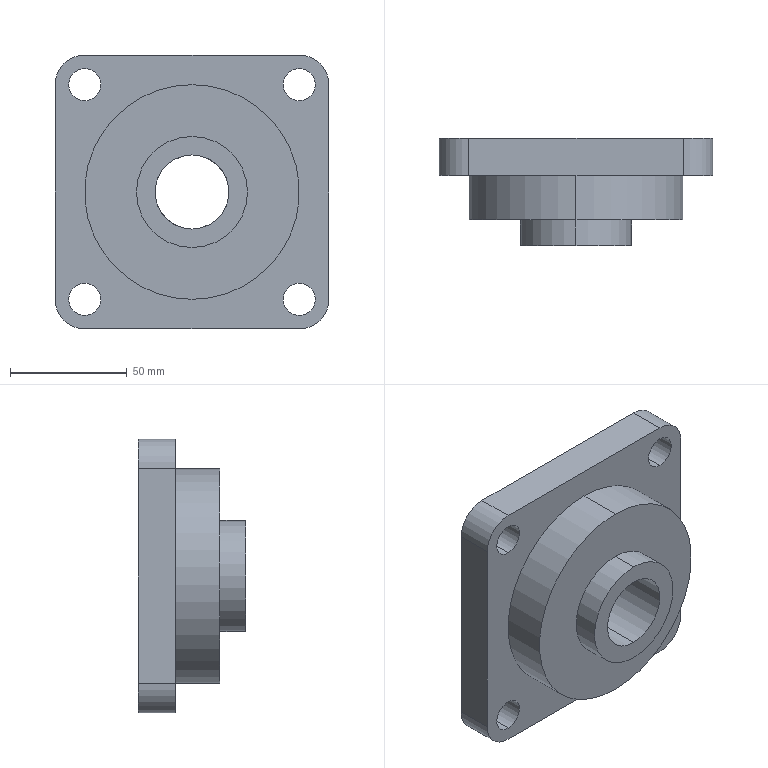Component | SolidWorks | LX-TSJ-02-1 | 1 solid | 26 faces | box 117.48 x 46.04 x 117.48 mm | volume 317559 mm3 | cylinder 18 | plane 8 | commonest cylinder face diameters 13.811 x8 25.4 x4 31.75 x2 92.075 x2 47.625 x2
STEP:
#1=COLOUR_RGB('',0.7922,0.8196,0.9333);
#2=FILL_AREA_STYLE_COLOUR('',#1);
#3=FILL_AREA_STYLE('',(#2));
#4=SURFACE_STYLE_FILL_AREA(#3);
#5=SURFACE_SIDE_STYLE('',(#4));
#6=SURFACE_STYLE_USAGE(.BOTH.,#5);
#7=PRESENTATION_STYLE_ASSIGNMENT((#6));
#8=CARTESIAN_POINT('',(-4.843,-15.157,-15.686));
#9=VERTEX_POINT('',#8);
#10=CARTESIAN_POINT('',(-4.843,-15.157,-16.936));
#11=VERTEX_POINT('',#10);
#12=CARTESIAN_POINT('',(-4.843,-15.157,-15.686));
#13=CARTESIAN_POINT('',(-4.926,-15.157,-15.686));
#14=CARTESIAN_POINT('',(-5.006,-15.157,-15.702));
#15=CARTESIAN_POINT('',(-5.159,-15.157,-15.765));
#16=CARTESIAN_POINT('',(-5.227,-15.157,-15.81));
#17=CARTESIAN_POINT('',(-5.344,-15.157,-15.928));
#18=CARTESIAN_POINT('',(-5.389,-15.157,-15.995));
#19=CARTESIAN_POINT('',(-5.453,-15.157,-16.148));
#20=CARTESIAN_POINT('',(-5.468,-15.157,-16.228));
#21=CARTESIAN_POINT('',(-5.468,-15.157,-16.394));
#22=CARTESIAN_POINT('',(-5.453,-15.157,-16.474));
#23=CARTESIAN_POINT('',(-5.389,-15.157,-16.627));
#24=CARTESIAN_POINT('',(-5.344,-15.157,-16.694));
#25=CARTESIAN_POINT('',(-5.227,-15.157,-16.811));
#26=CARTESIAN_POINT('',(-5.159,-15.157,-16.857));
#27=CARTESIAN_POINT('',(-5.006,-15.157,-16.92));
#28=CARTESIAN_POINT('',(-4.926,-15.157,-16.936));
#29=CARTESIAN_POINT('',(-4.843,-15.157,-16.936));
#30=B_SPLINE_CURVE_WITH_KNOTS('',3,(#12,#13,#14,#15,#16,#17,#18,#19,#20,#21,#22,#23,#24,#25,#26,#27,#28,#29),.UNSPECIFIED.,.F.,.F.,(4,2,2,2,2,2,2,2,4),(0.5,0.5625,0.625,0.6875,0.75,0.8125,0.875,0.9375,1.),.UNSPECIFIED.);
#31=EDGE_CURVE('',#9,#11,#30,.T.);
#32=ORIENTED_EDGE('',*,*,#31,.F.);
#33=CARTESIAN_POINT('',(-4.843,-16.969,-15.686));
#34=VERTEX_POINT('',#33);
#35=CARTESIAN_POINT('',(-4.843,-16.969,-15.686));
#36=DIRECTION('',(0.,-1.,-0.));
#37=VECTOR('',#36,39.37);
#38=LINE('',#35,#37);
#39=EDGE_CURVE('',#9,#34,#38,.T.);
#40=ORIENTED_EDGE('',*,*,#39,.T.);
#41=CARTESIAN_POINT('',(-4.843,-16.969,-16.936));
#42=VERTEX_POINT('',#41);
#43=CARTESIAN_POINT('',(-4.843,-16.969,-16.311));
#44=DIRECTION('',(0.,-1.,-0.));
#45=DIRECTION('',(0.,0.,-1.));
#46=AXIS2_PLACEMENT_3D('',#43,#44,#45);
#47=CIRCLE('',#46,0.625);
#48=EDGE_CURVE('',#34,#42,#47,.T.);
#49=ORIENTED_EDGE('',*,*,#48,.T.);
#50=CARTESIAN_POINT('',(-4.843,-16.969,-16.936));
#51=DIRECTION('',(0.,-1.,-0.));
#52=VECTOR('',#51,39.37);
#53=LINE('',#50,#52);
#54=EDGE_CURVE('',#11,#42,#53,.T.);
#55=ORIENTED_EDGE('',*,*,#54,.F.);
#56=EDGE_LOOP('',(#32,#40,#49,#55));
#57=FACE_OUTER_BOUND('',#56,.T.);
#58=CARTESIAN_POINT('',(-4.843,-16.969,-16.311));
#59=DIRECTION('',(0.,-1.,-0.));
#60=DIRECTION('',(0.,0.,-1.));
#61=AXIS2_PLACEMENT_3D('',#58,#59,#60);
#62=CYLINDRICAL_SURFACE('',#61,0.625);
#63=ADVANCED_FACE('',(#57),#62,.F.);
#64=CARTESIAN_POINT('',(-4.843,-16.532,-14.498));
#65=VERTEX_POINT('',#64);
#66=CARTESIAN_POINT('',(-4.843,-16.532,-18.123));
#67=VERTEX_POINT('',#66);
#68=CARTESIAN_POINT('',(-4.843,-16.532,-16.311));
#69=DIRECTION('',(-0.,1.,0.));
#70=DIRECTION('',(-0.,-0.,1.));
#71=AXIS2_PLACEMENT_3D('',#68,#69,#70);
#72=CIRCLE('',#71,1.813);
#73=EDGE_CURVE('',#65,#67,#72,.T.);
#74=ORIENTED_EDGE('',*,*,#73,.T.);
#75=CARTESIAN_POINT('',(-4.843,-15.782,-18.123));
#76=VERTEX_POINT('',#75);
#77=CARTESIAN_POINT('',(-4.843,-16.532,-18.123));
#78=DIRECTION('',(-0.,1.,0.));
#79=VECTOR('',#78,39.37);
#80=LINE('',#77,#79);
#81=EDGE_CURVE('',#67,#76,#80,.T.);
#82=ORIENTED_EDGE('',*,*,#81,.T.);
#83=CARTESIAN_POINT('',(-4.843,-15.782,-14.498));
#84=VERTEX_POINT('',#83);
#85=CARTESIAN_POINT('',(-4.843,-15.782,-16.311));
#86=DIRECTION('',(-0.,1.,0.));
#87=DIRECTION('',(-0.,-0.,1.));
#88=AXIS2_PLACEMENT_3D('',#85,#86,#87);
#89=CIRCLE('',#88,1.813);
#90=EDGE_CURVE('',#84,#76,#89,.T.);
#91=ORIENTED_EDGE('',*,*,#90,.F.);
#92=CARTESIAN_POINT('',(-4.843,-16.532,-14.498));
#93=DIRECTION('',(-0.,1.,0.));
#94=VECTOR('',#93,39.37);
#95=LINE('',#92,#94);
#96=EDGE_CURVE('',#65,#84,#95,.T.);
#97=ORIENTED_EDGE('',*,*,#96,.F.);
#98=EDGE_LOOP('',(#74,#82,#91,#97));
#99=FACE_OUTER_BOUND('',#98,.T.);
#100=CARTESIAN_POINT('',(-4.843,-16.532,-16.311));
#101=DIRECTION('',(-0.,1.,0.));
#102=DIRECTION('',(-0.,-0.,1.));
#103=AXIS2_PLACEMENT_3D('',#100,#101,#102);
#104=CYLINDRICAL_SURFACE('',#103,1.813);
#105=ADVANCED_FACE('',(#99),#104,.T.);
#106=CARTESIAN_POINT('',(-6.656,-15.157,-14.77));
#107=VERTEX_POINT('',#106);
#108=CARTESIAN_POINT('',(-6.656,-15.157,-14.227));
#109=VERTEX_POINT('',#108);
#110=CARTESIAN_POINT('',(-6.656,-15.157,-14.498));
#111=DIRECTION('',(-0.,1.,0.));
#112=DIRECTION('',(0.,0.,-1.));
#113=AXIS2_PLACEMENT_3D('',#110,#111,#112);
#114=CIRCLE('',#113,0.2719);
#115=EDGE_CURVE('',#107,#109,#114,.T.);
#116=ORIENTED_EDGE('',*,*,#115,.T.);
#117=CARTESIAN_POINT('',(-6.656,-15.782,-14.227));
#118=VERTEX_POINT('',#117);
#119=CARTESIAN_POINT('',(-6.656,-15.782,-14.227));
#120=DIRECTION('',(0.,-1.,-0.));
#121=VECTOR('',#120,39.37);
#122=LINE('',#119,#121);
#123=EDGE_CURVE('',#109,#118,#122,.T.);
#124=ORIENTED_EDGE('',*,*,#123,.T.);
#125=CARTESIAN_POINT('',(-6.656,-15.782,-14.77));
#126=VERTEX_POINT('',#125);
#127=CARTESIAN_POINT('',(-6.656,-15.782,-14.498));
#128=DIRECTION('',(-0.,1.,0.));
#129=DIRECTION('',(0.,0.,-1.));
#130=AXIS2_PLACEMENT_3D('',#127,#128,#129);
#131=CIRCLE('',#130,0.2719);
#132=EDGE_CURVE('',#126,#118,#131,.T.);
#133=ORIENTED_EDGE('',*,*,#132,.F.);
#134=CARTESIAN_POINT('',(-6.656,-15.782,-14.77));
#135=DIRECTION('',(0.,-1.,-0.));
#136=VECTOR('',#135,39.37);
#137=LINE('',#134,#136);
#138=EDGE_CURVE('',#107,#126,#137,.T.);
#139=ORIENTED_EDGE('',*,*,#138,.F.);
#140=EDGE_LOOP('',(#116,#124,#133,#139));
#141=FACE_OUTER_BOUND('',#140,.T.);
#142=CARTESIAN_POINT('',(-6.656,-15.782,-14.498));
#143=DIRECTION('',(0.,-1.,-0.));
#144=DIRECTION('',(0.,0.,-1.));
#145=AXIS2_PLACEMENT_3D('',#142,#143,#144);
#146=CYLINDRICAL_SURFACE('',#145,0.2719);
#147=ADVANCED_FACE('',(#141),#146,.F.);
#148=CARTESIAN_POINT('',(-6.656,-15.157,-18.395));
#149=VERTEX_POINT('',#148);
#150=CARTESIAN_POINT('',(-6.656,-15.157,-17.852));
#151=VERTEX_POINT('',#150);
#152=CARTESIAN_POINT('',(-6.656,-15.157,-18.123));
#153=DIRECTION('',(-0.,1.,0.));
#154=DIRECTION('',(0.,0.,-1.));
#155=AXIS2_PLACEMENT_3D('',#152,#153,#154);
#156=CIRCLE('',#155,0.2719);
#157=EDGE_CURVE('',#149,#151,#156,.T.);
#158=ORIENTED_EDGE('',*,*,#157,.T.);
#159=CARTESIAN_POINT('',(-6.656,-15.782,-17.852));
#160=VERTEX_POINT('',#159);
#161=CARTESIAN_POINT('',(-6.656,-15.782,-17.852));
#162=DIRECTION('',(0.,-1.,-0.));
#163=VECTOR('',#162,39.37);
#164=LINE('',#161,#163);
#165=EDGE_CURVE('',#151,#160,#164,.T.);
#166=ORIENTED_EDGE('',*,*,#165,.T.);
#167=CARTESIAN_POINT('',(-6.656,-15.782,-18.395));
#168=VERTEX_POINT('',#167);
#169=CARTESIAN_POINT('',(-6.656,-15.782,-18.123));
#170=DIRECTION('',(-0.,1.,0.));
#171=DIRECTION('',(0.,0.,-1.));
#172=AXIS2_PLACEMENT_3D('',#169,#170,#171);
#173=CIRCLE('',#172,0.2719);
#174=EDGE_CURVE('',#168,#160,#173,.T.);
#175=ORIENTED_EDGE('',*,*,#174,.F.);
#176=CARTESIAN_POINT('',(-6.656,-15.782,-18.395));
#177=DIRECTION('',(0.,-1.,-0.));
#178=VECTOR('',#177,39.37);
#179=LINE('',#176,#178);
#180=EDGE_CURVE('',#149,#168,#179,.T.);
#181=ORIENTED_EDGE('',*,*,#180,.F.);
#182=EDGE_LOOP('',(#158,#166,#175,#181));
#183=FACE_OUTER_BOUND('',#182,.T.);
#184=CARTESIAN_POINT('',(-6.656,-15.782,-18.123));
#185=DIRECTION('',(0.,-1.,-0.));
#186=DIRECTION('',(0.,0.,-1.));
#187=AXIS2_PLACEMENT_3D('',#184,#185,#186);
#188=CYLINDRICAL_SURFACE('',#187,0.2719);
#189=ADVANCED_FACE('',(#183),#188,.F.);
#190=CARTESIAN_POINT('',(-3.031,-15.157,-14.77));
#191=VERTEX_POINT('',#190);
#192=CARTESIAN_POINT('',(-3.031,-15.157,-14.227));
#193=VERTEX_POINT('',#192);
#194=CARTESIAN_POINT('',(-3.031,-15.157,-14.498));
#195=DIRECTION('',(-0.,1.,0.));
#196=DIRECTION('',(0.,0.,-1.));
#197=AXIS2_PLACEMENT_3D('',#194,#195,#196);
#198=CIRCLE('',#197,0.2719);
#199=EDGE_CURVE('',#191,#193,#198,.T.);
#200=ORIENTED_EDGE('',*,*,#199,.T.);
#201=CARTESIAN_POINT('',(-3.031,-15.782,-14.227));
#202=VERTEX_POINT('',#201);
#203=CARTESIAN_POINT('',(-3.031,-15.782,-14.227));
#204=DIRECTION('',(0.,-1.,-0.));
#205=VECTOR('',#204,39.37);
#206=LINE('',#203,#205);
#207=EDGE_CURVE('',#193,#202,#206,.T.);
#208=ORIENTED_EDGE('',*,*,#207,.T.);
#209=CARTESIAN_POINT('',(-3.031,-15.782,-14.77));
#210=VERTEX_POINT('',#209);
#211=CARTESIAN_POINT('',(-3.031,-15.782,-14.498));
#212=DIRECTION('',(-0.,1.,0.));
#213=DIRECTION('',(0.,0.,-1.));
#214=AXIS2_PLACEMENT_3D('',#211,#212,#213);
#215=CIRCLE('',#214,0.2719);
#216=EDGE_CURVE('',#210,#202,#215,.T.);
#217=ORIENTED_EDGE('',*,*,#216,.F.);
#218=CARTESIAN_POINT('',(-3.031,-15.782,-14.77));
#219=DIRECTION('',(0.,-1.,-0.));
#220=VECTOR('',#219,39.37);
#221=LINE('',#218,#220);
#222=EDGE_CURVE('',#191,#210,#221,.T.);
#223=ORIENTED_EDGE('',*,*,#222,.F.);
#224=EDGE_LOOP('',(#200,#208,#217,#223));
#225=FACE_OUTER_BOUND('',#224,.T.);
#226=CARTESIAN_POINT('',(-3.031,-15.782,-14.498));
#227=DIRECTION('',(0.,-1.,-0.));
#228=DIRECTION('',(0.,0.,-1.));
#229=AXIS2_PLACEMENT_3D('',#226,#227,#228);
#230=CYLINDRICAL_SURFACE('',#229,0.2719);
#231=ADVANCED_FACE('',(#225),#230,.F.);
#232=CARTESIAN_POINT('',(-3.031,-15.157,-18.395));
#233=VERTEX_POINT('',#232);
#234=CARTESIAN_POINT('',(-3.031,-15.157,-17.852));
#235=VERTEX_POINT('',#234);
#236=CARTESIAN_POINT('',(-3.031,-15.157,-18.123));
#237=DIRECTION('',(-0.,1.,0.));
#238=DIRECTION('',(0.,0.,-1.));
#239=AXIS2_PLACEMENT_3D('',#236,#237,#238);
#240=CIRCLE('',#239,0.2719);
#241=EDGE_CURVE('',#233,#235,#240,.T.);
#242=ORIENTED_EDGE('',*,*,#241,.T.);
#243=CARTESIAN_POINT('',(-3.031,-15.782,-17.852));
#244=VERTEX_POINT('',#243);
#245=CARTESIAN_POINT('',(-3.031,-15.782,-17.852));
#246=DIRECTION('',(0.,-1.,-0.));
#247=VECTOR('',#246,39.37);
#248=LINE('',#245,#247);
#249=EDGE_CURVE('',#235,#244,#248,.T.);
#250=ORIENTED_EDGE('',*,*,#249,.T.);
#251=CARTESIAN_POINT('',(-3.031,-15.782,-18.395));
#252=VERTEX_POINT('',#251);
#253=CARTESIAN_POINT('',(-3.031,-15.782,-18.123));
#254=DIRECTION('',(-0.,1.,0.));
#255=DIRECTION('',(0.,0.,-1.));
#256=AXIS2_PLACEMENT_3D('',#253,#254,#255);
#257=CIRCLE('',#256,0.2719);
#258=EDGE_CURVE('',#252,#244,#257,.T.);
#259=ORIENTED_EDGE('',*,*,#258,.F.);
#260=CARTESIAN_POINT('',(-3.031,-15.782,-18.395));
#261=DIRECTION('',(0.,-1.,-0.));
#262=VECTOR('',#261,39.37);
#263=LINE('',#260,#262);
#264=EDGE_CURVE('',#233,#252,#263,.T.);
#265=ORIENTED_EDGE('',*,*,#264,.F.);
#266=EDGE_LOOP('',(#242,#250,#259,#265));
#267=FACE_OUTER_BOUND('',#266,.T.);
#268=CARTESIAN_POINT('',(-3.031,-15.782,-18.123));
#269=DIRECTION('',(0.,-1.,-0.));
#270=DIRECTION('',(0.,0.,-1.));
#271=AXIS2_PLACEMENT_3D('',#268,#269,#270);
#272=CYLINDRICAL_SURFACE('',#271,0.2719);
#273=ADVANCED_FACE('',(#267),#272,.F.);
#274=CARTESIAN_POINT('',(-4.843,-16.969,-17.248));
#275=VERTEX_POINT('',#274);
#276=CARTESIAN_POINT('',(-4.843,-16.969,-15.373));
#277=VERTEX_POINT('',#276);
#278=CARTESIAN_POINT('',(-4.843,-16.969,-16.311));
#279=DIRECTION('',(0.,-1.,-0.));
#280=DIRECTION('',(0.,0.,-1.));
#281=AXIS2_PLACEMENT_3D('',#278,#279,#280);
#282=CIRCLE('',#281,0.9375);
#283=EDGE_CURVE('',#275,#277,#282,.T.);
#284=ORIENTED_EDGE('',*,*,#283,.F.);
#285=CARTESIAN_POINT('',(-4.843,-16.532,-17.248));
#286=VERTEX_POINT('',#285);
#287=CARTESIAN_POINT('',(-4.843,-16.969,-17.248));
#288=DIRECTION('',(-0.,1.,0.));
#289=VECTOR('',#288,39.37);
#290=LINE('',#287,#289);
#291=EDGE_CURVE('',#275,#286,#290,.T.);
#292=ORIENTED_EDGE('',*,*,#291,.T.);
#293=CARTESIAN_POINT('',(-4.843,-16.532,-15.373));
#294=VERTEX_POINT('',#293);
#295=CARTESIAN_POINT('',(-4.843,-16.532,-16.311));
#296=DIRECTION('',(-0.,1.,0.));
#297=DIRECTION('',(0.,0.,-1.));
#298=AXIS2_PLACEMENT_3D('',#295,#296,#297);
#299=CIRCLE('',#298,0.9375);
#300=EDGE_CURVE('',#294,#286,#299,.T.);
#301=ORIENTED_EDGE('',*,*,#300,.F.);
#302=CARTESIAN_POINT('',(-4.843,-16.969,-15.373));
#303=DIRECTION('',(-0.,1.,0.));
#304=VECTOR('',#303,39.37);
#305=LINE('',#302,#304);
#306=EDGE_CURVE('',#277,#294,#305,.T.);
#307=ORIENTED_EDGE('',*,*,#306,.F.);
#308=EDGE_LOOP('',(#284,#292,#301,#307));
#309=FACE_OUTER_BOUND('',#308,.T.);
#310=CARTESIAN_POINT('',(-4.843,-16.969,-16.311));
#311=DIRECTION('',(-0.,1.,0.));
#312=DIRECTION('',(0.,-0.,1.));
#313=AXIS2_PLACEMENT_3D('',#310,#311,#312);
#314=CYLINDRICAL_SURFACE('',#313,0.9375);
#315=ADVANCED_FACE('',(#309),#314,.T.);
#316=ORIENTED_EDGE('',*,*,#291,.F.);
#317=CARTESIAN_POINT('',(-4.843,-16.969,-16.311));
#318=DIRECTION('',(0.,-1.,-0.));
#319=DIRECTION('',(0.,0.,-1.));
#320=AXIS2_PLACEMENT_3D('',#317,#318,#319);
#321=CIRCLE('',#320,0.9375);
#322=EDGE_CURVE('',#277,#275,#321,.T.);
#323=ORIENTED_EDGE('',*,*,#322,.F.);
#324=ORIENTED_EDGE('',*,*,#306,.T.);
#325=CARTESIAN_POINT('',(-4.843,-16.532,-16.311));
#326=DIRECTION('',(-0.,1.,0.));
#327=DIRECTION('',(0.,0.,-1.));
#328=AXIS2_PLACEMENT_3D('',#325,#326,#327);
#329=CIRCLE('',#328,0.9375);
#330=EDGE_CURVE('',#286,#294,#329,.T.);
#331=ORIENTED_EDGE('',*,*,#330,.F.);
#332=EDGE_LOOP('',(#316,#323,#324,#331));
#333=FACE_OUTER_BOUND('',#332,.T.);
#334=CARTESIAN_POINT('',(-4.843,-16.969,-16.311));
#335=DIRECTION('',(-0.,1.,0.));
#336=DIRECTION('',(0.,-0.,1.));
#337=AXIS2_PLACEMENT_3D('',#334,#335,#336);
#338=CYLINDRICAL_SURFACE('',#337,0.9375);
#339=ADVANCED_FACE('',(#333),#338,.T.);
#340=CARTESIAN_POINT('',(-4.843,-15.157,-16.936));
#341=CARTESIAN_POINT('',(-4.761,-15.157,-16.936));
#342=CARTESIAN_POINT('',(-4.681,-15.157,-16.92));
#343=CARTESIAN_POINT('',(-4.528,-15.157,-16.857));
#344=CARTESIAN_POINT('',(-4.46,-15.157,-16.811));
#345=CARTESIAN_POINT('',(-4.343,-15.157,-16.694));
#346=CARTESIAN_POINT('',(-4.298,-15.157,-16.627));
#347=CARTESIAN_POINT('',(-4.234,-15.157,-16.474));
#348=CARTESIAN_POINT('',(-4.218,-15.157,-16.394));
#349=CARTESIAN_POINT('',(-4.218,-15.157,-16.228));
#350=CARTESIAN_POINT('',(-4.234,-15.157,-16.148));
#351=CARTESIAN_POINT('',(-4.298,-15.157,-15.995));
#352=CARTESIAN_POINT('',(-4.343,-15.157,-15.928));
#353=CARTESIAN_POINT('',(-4.46,-15.157,-15.81));
#354=CARTESIAN_POINT('',(-4.528,-15.157,-15.765));
#355=CARTESIAN_POINT('',(-4.681,-15.157,-15.702));
#356=CARTESIAN_POINT('',(-4.761,-15.157,-15.686));
#357=CARTESIAN_POINT('',(-4.843,-15.157,-15.686));
#358=B_SPLINE_CURVE_WITH_KNOTS('',3,(#340,#341,#342,#343,#344,#345,#346,#347,#348,#349,#350,#351,#352,#353,#354,#355,#356,#357),.UNSPECIFIED.,.F.,.F.,(4,2,2,2,2,2,2,2,4),(0.,0.0625,0.125,0.1875,0.25,0.3125,0.375,0.4375,0.5),.UNSPECIFIED.);
#359=EDGE_CURVE('',#11,#9,#358,.T.);
#360=ORIENTED_EDGE('',*,*,#359,.T.);
#361=ORIENTED_EDGE('',*,*,#31,.T.);
#362=EDGE_LOOP('',(#360,#361));
#363=FACE_BOUND('',#362,.T.);
#364=CARTESIAN_POINT('',(-3.031,-15.157,-18.623));
#365=VERTEX_POINT('',#364);
#366=CARTESIAN_POINT('',(-2.531,-15.157,-18.123));
#367=VERTEX_POINT('',#366);
#368=CARTESIAN_POINT('',(-3.031,-15.157,-18.123));
#369=DIRECTION('',(0.,-1.,-0.));
#370=DIRECTION('',(0.,0.,-1.));
#371=AXIS2_PLACEMENT_3D('',#368,#369,#370);
#372=CIRCLE('',#371,0.5);
#373=EDGE_CURVE('',#365,#367,#372,.T.);
#374=ORIENTED_EDGE('',*,*,#373,.F.);
#375=CARTESIAN_POINT('',(-6.656,-15.157,-18.623));
#376=VERTEX_POINT('',#375);
#377=CARTESIAN_POINT('',(-7.156,-15.157,-18.623));
#378=DIRECTION('',(1.,0.,0.));
#379=VECTOR('',#378,39.37);
#380=LINE('',#377,#379);
#381=EDGE_CURVE('',#376,#365,#380,.T.);
#382=ORIENTED_EDGE('',*,*,#381,.F.);
#383=CARTESIAN_POINT('',(-7.156,-15.157,-18.123));
#384=VERTEX_POINT('',#383);
#385=CARTESIAN_POINT('',(-6.656,-15.157,-18.123));
#386=DIRECTION('',(0.,-1.,-0.));
#387=DIRECTION('',(0.,-0.,1.));
#388=AXIS2_PLACEMENT_3D('',#385,#386,#387);
#389=CIRCLE('',#388,0.5);
#390=EDGE_CURVE('',#384,#376,#389,.T.);
#391=ORIENTED_EDGE('',*,*,#390,.F.);
#392=CARTESIAN_POINT('',(-7.156,-15.157,-14.498));
#393=VERTEX_POINT('',#392);
#394=CARTESIAN_POINT('',(-7.156,-15.157,-18.623));
#395=DIRECTION('',(0.,0.,-1.));
#396=VECTOR('',#395,39.37);
#397=LINE('',#394,#396);
#398=EDGE_CURVE('',#393,#384,#397,.T.);
#399=ORIENTED_EDGE('',*,*,#398,.F.);
#400=CARTESIAN_POINT('',(-6.656,-15.157,-13.998));
#401=VERTEX_POINT('',#400);
#402=CARTESIAN_POINT('',(-6.656,-15.157,-14.498));
#403=DIRECTION('',(0.,-1.,-0.));
#404=DIRECTION('',(0.,0.,-1.));
#405=AXIS2_PLACEMENT_3D('',#402,#403,#404);
#406=CIRCLE('',#405,0.5);
#407=EDGE_CURVE('',#401,#393,#406,.T.);
#408=ORIENTED_EDGE('',*,*,#407,.F.);
#409=CARTESIAN_POINT('',(-3.031,-15.157,-13.998));
#410=VERTEX_POINT('',#409);
#411=CARTESIAN_POINT('',(-7.156,-15.157,-13.998));
#412=DIRECTION('',(-1.,-0.,-0.));
#413=VECTOR('',#412,39.37);
#414=LINE('',#411,#413);
#415=EDGE_CURVE('',#410,#401,#414,.T.);
#416=ORIENTED_EDGE('',*,*,#415,.F.);
#417=CARTESIAN_POINT('',(-2.531,-15.157,-14.498));
#418=VERTEX_POINT('',#417);
#419=CARTESIAN_POINT('',(-3.031,-15.157,-14.498));
#420=DIRECTION('',(0.,-1.,-0.));
#421=DIRECTION('',(0.,0.,-1.));
#422=AXIS2_PLACEMENT_3D('',#419,#420,#421);
#423=CIRCLE('',#422,0.5);
#424=EDGE_CURVE('',#418,#410,#423,.T.);
#425=ORIENTED_EDGE('',*,*,#424,.F.);
#426=CARTESIAN_POINT('',(-2.531,-15.157,-18.623));
#427=DIRECTION('',(-0.,-0.,1.));
#428=VECTOR('',#427,39.37);
#429=LINE('',#426,#428);
#430=EDGE_CURVE('',#367,#418,#429,.T.);
#431=ORIENTED_EDGE('',*,*,#430,.F.);
#432=EDGE_LOOP('',(#374,#382,#391,#399,#408,#416,#425,#431));
#433=FACE_OUTER_BOUND('',#432,.T.);
#434=ORIENTED_EDGE('',*,*,#115,.F.);
#435=CARTESIAN_POINT('',(-6.656,-15.157,-14.498));
#436=DIRECTION('',(-0.,1.,0.));
#437=DIRECTION('',(0.,0.,-1.));
#438=AXIS2_PLACEMENT_3D('',#435,#436,#437);
#439=CIRCLE('',#438,0.2719);
#440=EDGE_CURVE('',#109,#107,#439,.T.);
#441=ORIENTED_EDGE('',*,*,#440,.F.);
#442=EDGE_LOOP('',(#434,#441));
#443=FACE_BOUND('',#442,.T.);
#444=ORIENTED_EDGE('',*,*,#157,.F.);
#445=CARTESIAN_POINT('',(-6.656,-15.157,-18.123));
#446=DIRECTION('',(-0.,1.,0.));
#447=DIRECTION('',(0.,0.,-1.));
#448=AXIS2_PLACEMENT_3D('',#445,#446,#447);
#449=CIRCLE('',#448,0.2719);
#450=EDGE_CURVE('',#151,#149,#449,.T.);
#451=ORIENTED_EDGE('',*,*,#450,.F.);
#452=EDGE_LOOP('',(#444,#451));
#453=FACE_BOUND('',#452,.T.);
#454=ORIENTED_EDGE('',*,*,#199,.F.);
#455=CARTESIAN_POINT('',(-3.031,-15.157,-14.498));
#456=DIRECTION('',(-0.,1.,0.));
#457=DIRECTION('',(0.,0.,-1.));
#458=AXIS2_PLACEMENT_3D('',#455,#456,#457);
#459=CIRCLE('',#458,0.2719);
#460=EDGE_CURVE('',#193,#191,#459,.T.);
#461=ORIENTED_EDGE('',*,*,#460,.F.);
#462=EDGE_LOOP('',(#454,#461));
#463=FACE_BOUND('',#462,.T.);
#464=ORIENTED_EDGE('',*,*,#241,.F.);
#465=CARTESIAN_POINT('',(-3.031,-15.157,-18.123));
#466=DIRECTION('',(-0.,1.,0.));
#467=DIRECTION('',(0.,0.,-1.));
#468=AXIS2_PLACEMENT_3D('',#465,#466,#467);
#469=CIRCLE('',#468,0.2719);
#470=EDGE_CURVE('',#235,#233,#469,.T.);
#471=ORIENTED_EDGE('',*,*,#470,.F.);
#472=EDGE_LOOP('',(#464,#471));
#473=FACE_BOUND('',#472,.T.);
#474=CARTESIAN_POINT('',(-7.156,-15.157,-18.623));
#475=DIRECTION('',(0.,-1.,-0.));
#476=DIRECTION('',(0.,0.,-1.));
#477=AXIS2_PLACEMENT_3D('',#474,#475,#476);
#478=PLANE('',#477);
#479=ADVANCED_FACE('',(#363,#433,#443,#453,#463,#473),#478,.F.);
#480=ORIENTED_EDGE('',*,*,#249,.F.);
#481=ORIENTED_EDGE('',*,*,#470,.T.);
#482=ORIENTED_EDGE('',*,*,#264,.T.);
#483=CARTESIAN_POINT('',(-3.031,-15.782,-18.123));
#484=DIRECTION('',(-0.,1.,0.));
#485=DIRECTION('',(0.,0.,-1.));
#486=AXIS2_PLACEMENT_3D('',#483,#484,#485);
#487=CIRCLE('',#486,0.2719);
#488=EDGE_CURVE('',#244,#252,#487,.T.);
#489=ORIENTED_EDGE('',*,*,#488,.F.);
#490=EDGE_LOOP('',(#480,#481,#482,#489));
#491=FACE_OUTER_BOUND('',#490,.T.);
#492=CARTESIAN_POINT('',(-3.031,-15.782,-18.123));
#493=DIRECTION('',(0.,-1.,-0.));
#494=DIRECTION('',(0.,0.,-1.));
#495=AXIS2_PLACEMENT_3D('',#492,#493,#494);
#496=CYLINDRICAL_SURFACE('',#495,0.2719);
#497=ADVANCED_FACE('',(#491),#496,.F.);
#498=ORIENTED_EDGE('',*,*,#207,.F.);
#499=ORIENTED_EDGE('',*,*,#460,.T.);
#500=ORIENTED_EDGE('',*,*,#222,.T.);
#501=CARTESIAN_POINT('',(-3.031,-15.782,-14.498));
#502=DIRECTION('',(-0.,1.,0.));
#503=DIRECTION('',(0.,0.,-1.));
#504=AXIS2_PLACEMENT_3D('',#501,#502,#503);
#505=CIRCLE('',#504,0.2719);
#506=EDGE_CURVE('',#202,#210,#505,.T.);
#507=ORIENTED_EDGE('',*,*,#506,.F.);
#508=EDGE_LOOP('',(#498,#499,#500,#507));
#509=FACE_OUTER_BOUND('',#508,.T.);
#510=CARTESIAN_POINT('',(-3.031,-15.782,-14.498));
#511=DIRECTION('',(0.,-1.,-0.));
#512=DIRECTION('',(0.,0.,-1.));
#513=AXIS2_PLACEMENT_3D('',#510,#511,#512);
#514=CYLINDRICAL_SURFACE('',#513,0.2719);
#515=ADVANCED_FACE('',(#509),#514,.F.);
#516=ORIENTED_EDGE('',*,*,#165,.F.);
#517=ORIENTED_EDGE('',*,*,#450,.T.);
#518=ORIENTED_EDGE('',*,*,#180,.T.);
#519=CARTESIAN_POINT('',(-6.656,-15.782,-18.123));
#520=DIRECTION('',(-0.,1.,0.));
#521=DIRECTION('',(0.,0.,-1.));
#522=AXIS2_PLACEMENT_3D('',#519,#520,#521);
#523=CIRCLE('',#522,0.2719);
#524=EDGE_CURVE('',#160,#168,#523,.T.);
#525=ORIENTED_EDGE('',*,*,#524,.F.);
#526=EDGE_LOOP('',(#516,#517,#518,#525));
#527=FACE_OUTER_BOUND('',#526,.T.);
#528=CARTESIAN_POINT('',(-6.656,-15.782,-18.123));
#529=DIRECTION('',(0.,-1.,-0.));
#530=DIRECTION('',(0.,0.,-1.));
#531=AXIS2_PLACEMENT_3D('',#528,#529,#530);
#532=CYLINDRICAL_SURFACE('',#531,0.2719);
#533=ADVANCED_FACE('',(#527),#532,.F.);
#534=ORIENTED_EDGE('',*,*,#123,.F.);
#535=ORIENTED_EDGE('',*,*,#440,.T.);
#536=ORIENTED_EDGE('',*,*,#138,.T.);
#537=CARTESIAN_POINT('',(-6.656,-15.782,-14.498));
#538=DIRECTION('',(-0.,1.,0.));
#539=DIRECTION('',(0.,0.,-1.));
#540=AXIS2_PLACEMENT_3D('',#537,#538,#539);
#541=CIRCLE('',#540,0.2719);
#542=EDGE_CURVE('',#118,#126,#541,.T.);
#543=ORIENTED_EDGE('',*,*,#542,.F.);
#544=EDGE_LOOP('',(#534,#535,#536,#543));
#545=FACE_OUTER_BOUND('',#544,.T.);
#546=CARTESIAN_POINT('',(-6.656,-15.782,-14.498));
#547=DIRECTION('',(0.,-1.,-0.));
#548=DIRECTION('',(0.,0.,-1.));
#549=AXIS2_PLACEMENT_3D('',#546,#547,#548);
#550=CYLINDRICAL_SURFACE('',#549,0.2719);
#551=ADVANCED_FACE('',(#545),#550,.F.);
#552=CARTESIAN_POINT('',(-7.156,-15.782,-14.498));
#553=VERTEX_POINT('',#552);
#554=CARTESIAN_POINT('',(-6.656,-15.782,-13.998));
#555=VERTEX_POINT('',#554);
#556=CARTESIAN_POINT('',(-6.656,-15.782,-14.498));
#557=DIRECTION('',(-0.,1.,0.));
#558=DIRECTION('',(0.,0.,-1.));
#559=AXIS2_PLACEMENT_3D('',#556,#557,#558);
#560=CIRCLE('',#559,0.5);
#561=EDGE_CURVE('',#553,#555,#560,.T.);
#562=ORIENTED_EDGE('',*,*,#561,.T.);
#563=CARTESIAN_POINT('',(-6.656,-15.157,-13.998));
#564=DIRECTION('',(-0.,1.,0.));
#565=VECTOR('',#564,39.37);
#566=LINE('',#563,#565);
#567=EDGE_CURVE('',#555,#401,#566,.T.);
#568=ORIENTED_EDGE('',*,*,#567,.T.);
#569=ORIENTED_EDGE('',*,*,#407,.T.);
#570=CARTESIAN_POINT('',(-7.156,-15.157,-14.498));
#571=DIRECTION('',(0.,-1.,-0.));
#572=VECTOR('',#571,39.37);
#573=LINE('',#570,#572);
#574=EDGE_CURVE('',#393,#553,#573,.T.);
#575=ORIENTED_EDGE('',*,*,#574,.T.);
#576=EDGE_LOOP('',(#562,#568,#569,#575));
#577=FACE_OUTER_BOUND('',#576,.T.);
#578=CARTESIAN_POINT('',(-6.656,-15.157,-14.498));
#579=DIRECTION('',(0.,-1.,-0.));
#580=DIRECTION('',(0.,0.,-1.));
#581=AXIS2_PLACEMENT_3D('',#578,#579,#580);
#582=CYLINDRICAL_SURFACE('',#581,0.5);
#583=ADVANCED_FACE('',(#577),#582,.T.);
#584=CARTESIAN_POINT('',(-3.031,-15.782,-13.998));
#585=VERTEX_POINT('',#584);
#586=CARTESIAN_POINT('',(-3.031,-15.157,-13.998));
#587=DIRECTION('',(0.,-1.,-0.));
#588=VECTOR('',#587,39.37);
#589=LINE('',#586,#588);
#590=EDGE_CURVE('',#410,#585,#589,.T.);
#591=ORIENTED_EDGE('',*,*,#590,.F.);
#592=ORIENTED_EDGE('',*,*,#415,.T.);
#593=ORIENTED_EDGE('',*,*,#567,.F.);
#594=CARTESIAN_POINT('',(-2.531,-15.782,-13.998));
#595=DIRECTION('',(-1.,-0.,-0.));
#596=VECTOR('',#595,39.37);
#597=LINE('',#594,#596);
#598=EDGE_CURVE('',#585,#555,#597,.T.);
#599=ORIENTED_EDGE('',*,*,#598,.F.);
#600=EDGE_LOOP('',(#591,#592,#593,#599));
#601=FACE_OUTER_BOUND('',#600,.T.);
#602=CARTESIAN_POINT('',(-2.531,-15.157,-13.998));
#603=DIRECTION('',(0.,0.,-1.));
#604=DIRECTION('',(1.,0.,0.));
#605=AXIS2_PLACEMENT_3D('',#602,#603,#604);
#606=PLANE('',#605);
#607=ADVANCED_FACE('',(#601),#606,.F.);
#608=CARTESIAN_POINT('',(-2.531,-15.782,-14.498));
#609=VERTEX_POINT('',#608);
#610=CARTESIAN_POINT('',(-3.031,-15.782,-14.498));
#611=DIRECTION('',(-0.,1.,0.));
#612=DIRECTION('',(0.,0.,-1.));
#613=AXIS2_PLACEMENT_3D('',#610,#611,#612);
#614=CIRCLE('',#613,0.5);
#615=EDGE_CURVE('',#585,#609,#614,.T.);
#616=ORIENTED_EDGE('',*,*,#615,.T.);
#617=CARTESIAN_POINT('',(-2.531,-15.157,-14.498));
#618=DIRECTION('',(-0.,1.,0.));
#619=VECTOR('',#618,39.37);
#620=LINE('',#617,#619);
#621=EDGE_CURVE('',#609,#418,#620,.T.);
#622=ORIENTED_EDGE('',*,*,#621,.T.);
#623=ORIENTED_EDGE('',*,*,#424,.T.);
#624=ORIENTED_EDGE('',*,*,#590,.T.);
#625=EDGE_LOOP('',(#616,#622,#623,#624));
#626=FACE_OUTER_BOUND('',#625,.T.);
#627=CARTESIAN_POINT('',(-3.031,-15.157,-14.498));
#628=DIRECTION('',(0.,-1.,-0.));
#629=DIRECTION('',(0.,0.,-1.));
#630=AXIS2_PLACEMENT_3D('',#627,#628,#629);
#631=CYLINDRICAL_SURFACE('',#630,0.5);
#632=ADVANCED_FACE('',(#626),#631,.T.);
#633=CARTESIAN_POINT('',(-2.531,-15.782,-18.123));
#634=VERTEX_POINT('',#633);
#635=CARTESIAN_POINT('',(-2.531,-15.157,-18.123));
#636=DIRECTION('',(0.,-1.,-0.));
#637=VECTOR('',#636,39.37);
#638=LINE('',#635,#637);
#639=EDGE_CURVE('',#367,#634,#638,.T.);
#640=ORIENTED_EDGE('',*,*,#639,.F.);
#641=ORIENTED_EDGE('',*,*,#430,.T.);
#642=ORIENTED_EDGE('',*,*,#621,.F.);
#643=CARTESIAN_POINT('',(-2.531,-15.782,-18.123));
#644=DIRECTION('',(-0.,-0.,1.));
#645=VECTOR('',#644,39.37);
#646=LINE('',#643,#645);
#647=EDGE_CURVE('',#634,#609,#646,.T.);
#648=ORIENTED_EDGE('',*,*,#647,.F.);
#649=EDGE_LOOP('',(#640,#641,#642,#648));
#650=FACE_OUTER_BOUND('',#649,.T.);
#651=CARTESIAN_POINT('',(-2.531,-15.157,-18.123));
#652=DIRECTION('',(-1.,-0.,-0.));
#653=DIRECTION('',(0.,0.,-1.));
#654=AXIS2_PLACEMENT_3D('',#651,#652,#653);
#655=PLANE('',#654);
#656=ADVANCED_FACE('',(#650),#655,.F.);
#657=CARTESIAN_POINT('',(-3.031,-15.782,-18.623));
#658=VERTEX_POINT('',#657);
#659=CARTESIAN_POINT('',(-3.031,-15.782,-18.123));
#660=DIRECTION('',(-0.,1.,0.));
#661=DIRECTION('',(-0.,0.,-1.));
#662=AXIS2_PLACEMENT_3D('',#659,#660,#661);
#663=CIRCLE('',#662,0.5);
#664=EDGE_CURVE('',#634,#658,#663,.T.);
#665=ORIENTED_EDGE('',*,*,#664,.T.);
#666=CARTESIAN_POINT('',(-3.031,-15.157,-18.623));
#667=DIRECTION('',(-0.,1.,0.));
#668=VECTOR('',#667,39.37);
#669=LINE('',#666,#668);
#670=EDGE_CURVE('',#658,#365,#669,.T.);
#671=ORIENTED_EDGE('',*,*,#670,.T.);
#672=ORIENTED_EDGE('',*,*,#373,.T.);
#673=ORIENTED_EDGE('',*,*,#639,.T.);
#674=EDGE_LOOP('',(#665,#671,#672,#673));
#675=FACE_OUTER_BOUND('',#674,.T.);
#676=CARTESIAN_POINT('',(-3.031,-15.157,-18.123));
#677=DIRECTION('',(0.,-1.,-0.));
#678=DIRECTION('',(0.,0.,-1.));
#679=AXIS2_PLACEMENT_3D('',#676,#677,#678);
#680=CYLINDRICAL_SURFACE('',#679,0.5);
#681=ADVANCED_FACE('',(#675),#680,.T.);
#682=ORIENTED_EDGE('',*,*,#670,.F.);
#683=CARTESIAN_POINT('',(-6.656,-15.782,-18.623));
#684=VERTEX_POINT('',#683);
#685=CARTESIAN_POINT('',(-7.156,-15.782,-18.623));
#686=DIRECTION('',(1.,0.,0.));
#687=VECTOR('',#686,39.37);
#688=LINE('',#685,#687);
#689=EDGE_CURVE('',#684,#658,#688,.T.);
#690=ORIENTED_EDGE('',*,*,#689,.F.);
#691=CARTESIAN_POINT('',(-6.656,-15.157,-18.623));
#692=DIRECTION('',(0.,-1.,-0.));
#693=VECTOR('',#692,39.37);
#694=LINE('',#691,#693);
#695=EDGE_CURVE('',#376,#684,#694,.T.);
#696=ORIENTED_EDGE('',*,*,#695,.F.);
#697=ORIENTED_EDGE('',*,*,#381,.T.);
#698=EDGE_LOOP('',(#682,#690,#696,#697));
#699=FACE_OUTER_BOUND('',#698,.T.);
#700=CARTESIAN_POINT('',(-7.156,-15.157,-18.623));
#701=DIRECTION('',(-0.,-0.,1.));
#702=DIRECTION('',(-1.,-0.,-0.));
#703=AXIS2_PLACEMENT_3D('',#700,#701,#702);
#704=PLANE('',#703);
#705=ADVANCED_FACE('',(#699),#704,.F.);
#706=ORIENTED_EDGE('',*,*,#390,.T.);
#707=ORIENTED_EDGE('',*,*,#695,.T.);
#708=CARTESIAN_POINT('',(-7.156,-15.782,-18.123));
#709=VERTEX_POINT('',#708);
#710=CARTESIAN_POINT('',(-6.656,-15.782,-18.123));
#711=DIRECTION('',(-0.,1.,0.));
#712=DIRECTION('',(0.,-0.,1.));
#713=AXIS2_PLACEMENT_3D('',#710,#711,#712);
#714=CIRCLE('',#713,0.5);
#715=EDGE_CURVE('',#684,#709,#714,.T.);
#716=ORIENTED_EDGE('',*,*,#715,.T.);
#717=CARTESIAN_POINT('',(-7.156,-15.157,-18.123));
#718=DIRECTION('',(-0.,1.,0.));
#719=VECTOR('',#718,39.37);
#720=LINE('',#717,#719);
#721=EDGE_CURVE('',#709,#384,#720,.T.);
#722=ORIENTED_EDGE('',*,*,#721,.T.);
#723=EDGE_LOOP('',(#706,#707,#716,#722));
#724=FACE_OUTER_BOUND('',#723,.T.);
#725=CARTESIAN_POINT('',(-6.656,-15.157,-18.123));
#726=DIRECTION('',(-0.,1.,0.));
#727=DIRECTION('',(0.,-0.,1.));
#728=AXIS2_PLACEMENT_3D('',#725,#726,#727);
#729=CYLINDRICAL_SURFACE('',#728,0.5);
#730=ADVANCED_FACE('',(#724),#729,.T.);
#731=ORIENTED_EDGE('',*,*,#574,.F.);
#732=ORIENTED_EDGE('',*,*,#398,.T.);
#733=ORIENTED_EDGE('',*,*,#721,.F.);
#734=CARTESIAN_POINT('',(-7.156,-15.782,-13.998));
#735=DIRECTION('',(0.,0.,-1.));
#736=VECTOR('',#735,39.37);
#737=LINE('',#734,#736);
#738=EDGE_CURVE('',#553,#709,#737,.T.);
#739=ORIENTED_EDGE('',*,*,#738,.F.);
#740=EDGE_LOOP('',(#731,#732,#733,#739));
#741=FACE_OUTER_BOUND('',#740,.T.);
#742=CARTESIAN_POINT('',(-7.156,-15.157,-13.998));
#743=DIRECTION('',(1.,0.,0.));
#744=DIRECTION('',(-0.,-0.,1.));
#745=AXIS2_PLACEMENT_3D('',#742,#743,#744);
#746=PLANE('',#745);
#747=ADVANCED_FACE('',(#741),#746,.F.);
#748=ORIENTED_EDGE('',*,*,#738,.T.);
#749=ORIENTED_EDGE('',*,*,#715,.F.);
#750=ORIENTED_EDGE('',*,*,#689,.T.);
#751=ORIENTED_EDGE('',*,*,#664,.F.);
#752=ORIENTED_EDGE('',*,*,#647,.T.);
#753=ORIENTED_EDGE('',*,*,#615,.F.);
#754=ORIENTED_EDGE('',*,*,#598,.T.);
#755=ORIENTED_EDGE('',*,*,#561,.F.);
#756=EDGE_LOOP('',(#748,#749,#750,#751,#752,#753,#754,#755));
#757=FACE_OUTER_BOUND('',#756,.T.);
#758=ORIENTED_EDGE('',*,*,#90,.T.);
#759=CARTESIAN_POINT('',(-4.843,-15.782,-16.311));
#760=DIRECTION('',(-0.,1.,0.));
#761=DIRECTION('',(-0.,-0.,1.));
#762=AXIS2_PLACEMENT_3D('',#759,#760,#761);
#763=CIRCLE('',#762,1.813);
#764=EDGE_CURVE('',#76,#84,#763,.T.);
#765=ORIENTED_EDGE('',*,*,#764,.T.);
#766=EDGE_LOOP('',(#758,#765));
#767=FACE_BOUND('',#766,.T.);
#768=ORIENTED_EDGE('',*,*,#132,.T.);
#769=ORIENTED_EDGE('',*,*,#542,.T.);
#770=EDGE_LOOP('',(#768,#769));
#771=FACE_BOUND('',#770,.T.);
#772=ORIENTED_EDGE('',*,*,#174,.T.);
#773=ORIENTED_EDGE('',*,*,#524,.T.);
#774=EDGE_LOOP('',(#772,#773));
#775=FACE_BOUND('',#774,.T.);
#776=ORIENTED_EDGE('',*,*,#216,.T.);
#777=ORIENTED_EDGE('',*,*,#506,.T.);
#778=EDGE_LOOP('',(#776,#777));
#779=FACE_BOUND('',#778,.T.);
#780=ORIENTED_EDGE('',*,*,#258,.T.);
#781=ORIENTED_EDGE('',*,*,#488,.T.);
#782=EDGE_LOOP('',(#780,#781));
#783=FACE_BOUND('',#782,.T.);
#784=CARTESIAN_POINT('',(-7.156,-15.782,-18.623));
#785=DIRECTION('',(0.,-1.,-0.));
#786=DIRECTION('',(0.,0.,-1.));
#787=AXIS2_PLACEMENT_3D('',#784,#785,#786);
#788=PLANE('',#787);
#789=ADVANCED_FACE('',(#757,#767,#771,#775,#779,#783),#788,.T.);
#790=ORIENTED_EDGE('',*,*,#81,.F.);
#791=CARTESIAN_POINT('',(-4.843,-16.532,-16.311));
#792=DIRECTION('',(-0.,1.,0.));
#793=DIRECTION('',(-0.,-0.,1.));
#794=AXIS2_PLACEMENT_3D('',#791,#792,#793);
#795=CIRCLE('',#794,1.813);
#796=EDGE_CURVE('',#67,#65,#795,.T.);
#797=ORIENTED_EDGE('',*,*,#796,.T.);
#798=ORIENTED_EDGE('',*,*,#96,.T.);
#799=ORIENTED_EDGE('',*,*,#764,.F.);
#800=EDGE_LOOP('',(#790,#797,#798,#799));
#801=FACE_OUTER_BOUND('',#800,.T.);
#802=CARTESIAN_POINT('',(-4.843,-16.532,-16.311));
#803=DIRECTION('',(-0.,1.,0.));
#804=DIRECTION('',(-0.,-0.,1.));
#805=AXIS2_PLACEMENT_3D('',#802,#803,#804);
#806=CYLINDRICAL_SURFACE('',#805,1.813);
#807=ADVANCED_FACE('',(#801),#806,.T.);
#808=ORIENTED_EDGE('',*,*,#73,.F.);
#809=ORIENTED_EDGE('',*,*,#796,.F.);
#810=EDGE_LOOP('',(#808,#809));
#811=FACE_OUTER_BOUND('',#810,.T.);
#812=ORIENTED_EDGE('',*,*,#300,.T.);
#813=ORIENTED_EDGE('',*,*,#330,.T.);
#814=EDGE_LOOP('',(#812,#813));
#815=FACE_BOUND('',#814,.T.);
#816=CARTESIAN_POINT('',(-3.031,-16.532,-16.311));
#817=DIRECTION('',(0.,-1.,-0.));
#818=DIRECTION('',(0.,0.,-1.));
#819=AXIS2_PLACEMENT_3D('',#816,#817,#818);
#820=PLANE('',#819);
#821=ADVANCED_FACE('',(#811,#815),#820,.T.);
#822=CARTESIAN_POINT('',(-4.843,-16.969,-16.311));
#823=DIRECTION('',(0.,-1.,-0.));
#824=DIRECTION('',(0.,0.,-1.));
#825=AXIS2_PLACEMENT_3D('',#822,#823,#824);
#826=CIRCLE('',#825,0.625);
#827=EDGE_CURVE('',#42,#34,#826,.T.);
#828=ORIENTED_EDGE('',*,*,#827,.F.);
#829=ORIENTED_EDGE('',*,*,#48,.F.);
#830=EDGE_LOOP('',(#828,#829));
#831=FACE_BOUND('',#830,.T.);
#832=ORIENTED_EDGE('',*,*,#322,.T.);
#833=ORIENTED_EDGE('',*,*,#283,.T.);
#834=EDGE_LOOP('',(#832,#833));
#835=FACE_OUTER_BOUND('',#834,.T.);
#836=CARTESIAN_POINT('',(-4.843,-16.969,-16.311));
#837=DIRECTION('',(0.,-1.,-0.));
#838=DIRECTION('',(0.,0.,-1.));
#839=AXIS2_PLACEMENT_3D('',#836,#837,#838);
#840=PLANE('',#839);
#841=ADVANCED_FACE('',(#831,#835),#840,.T.);
#842=ORIENTED_EDGE('',*,*,#39,.F.);
#843=ORIENTED_EDGE('',*,*,#359,.F.);
#844=ORIENTED_EDGE('',*,*,#54,.T.);
#845=ORIENTED_EDGE('',*,*,#827,.T.);
#846=EDGE_LOOP('',(#842,#843,#844,#845));
#847=FACE_OUTER_BOUND('',#846,.T.);
#848=CARTESIAN_POINT('',(-4.843,-16.969,-16.311));
#849=DIRECTION('',(0.,-1.,-0.));
#850=DIRECTION('',(0.,0.,-1.));
#851=AXIS2_PLACEMENT_3D('',#848,#849,#850);
#852=CYLINDRICAL_SURFACE('',#851,0.625);
#853=ADVANCED_FACE('',(#847),#852,.F.);
#854=CLOSED_SHELL('',(#63,#105,#147,#189,#231,#273,#315,#339,#479,#497,#515,#533,#551,#583,#607,#632,#656,#681,#705,#730,#747,#789,#807,#821,#841,#853));
#855=MANIFOLD_SOLID_BREP('',#854);
#856=STYLED_ITEM('',(#7),#855);
#857=(LENGTH_UNIT()NAMED_UNIT(*)SI_UNIT($,.METRE.));
#858=LENGTH_MEASURE_WITH_UNIT(LENGTH_MEASURE(0.0254),#857);
#859=DIMENSIONAL_EXPONENTS(1.,0.,0.,0.,0.,0.,0.);
#860=(CONVERSION_BASED_UNIT('',#858)LENGTH_UNIT()NAMED_UNIT(#859));
#861=UNCERTAINTY_MEASURE_WITH_UNIT(LENGTH_MEASURE(0.00001),#860,'','');
#862=(NAMED_UNIT(*)PLANE_ANGLE_UNIT()SI_UNIT($,.RADIAN.));
#863=(NAMED_UNIT(*)SI_UNIT($,.STERADIAN.)SOLID_ANGLE_UNIT());
#864=(GEOMETRIC_REPRESENTATION_CONTEXT(3)GLOBAL_UNCERTAINTY_ASSIGNED_CONTEXT((#861))GLOBAL_UNIT_ASSIGNED_CONTEXT((#860,#862,#863))REPRESENTATION_CONTEXT('',''));
#865=MECHANICAL_DESIGN_GEOMETRIC_PRESENTATION_REPRESENTATION('',(#856),#864);
#866=PRESENTATION_LAYER_ASSIGNMENT('','',(#856));
#867=CARTESIAN_POINT('',(0.,0.,0.));
#868=DIRECTION('',(0.,0.,1.));
#869=DIRECTION('',(1.,0.,0.));
#870=AXIS2_PLACEMENT_3D('',#867,#868,#869);
#871=(LENGTH_UNIT()NAMED_UNIT(*)SI_UNIT($,.METRE.));
#872=LENGTH_MEASURE_WITH_UNIT(LENGTH_MEASURE(0.0254),#871);
#873=DIMENSIONAL_EXPONENTS(1.,0.,0.,0.,0.,0.,0.);
#874=(CONVERSION_BASED_UNIT('',#872)LENGTH_UNIT()NAMED_UNIT(#873));
#875=UNCERTAINTY_MEASURE_WITH_UNIT(LENGTH_MEASURE(0.00001),#874,'','');
#876=(NAMED_UNIT(*)PLANE_ANGLE_UNIT()SI_UNIT($,.RADIAN.));
#877=(NAMED_UNIT(*)SI_UNIT($,.STERADIAN.)SOLID_ANGLE_UNIT());
#878=(GEOMETRIC_REPRESENTATION_CONTEXT(3)GLOBAL_UNCERTAINTY_ASSIGNED_CONTEXT((#875))GLOBAL_UNIT_ASSIGNED_CONTEXT((#874,#876,#877))REPRESENTATION_CONTEXT('',''));
#879=ADVANCED_BREP_SHAPE_REPRESENTATION('',(#855,#870),#878);